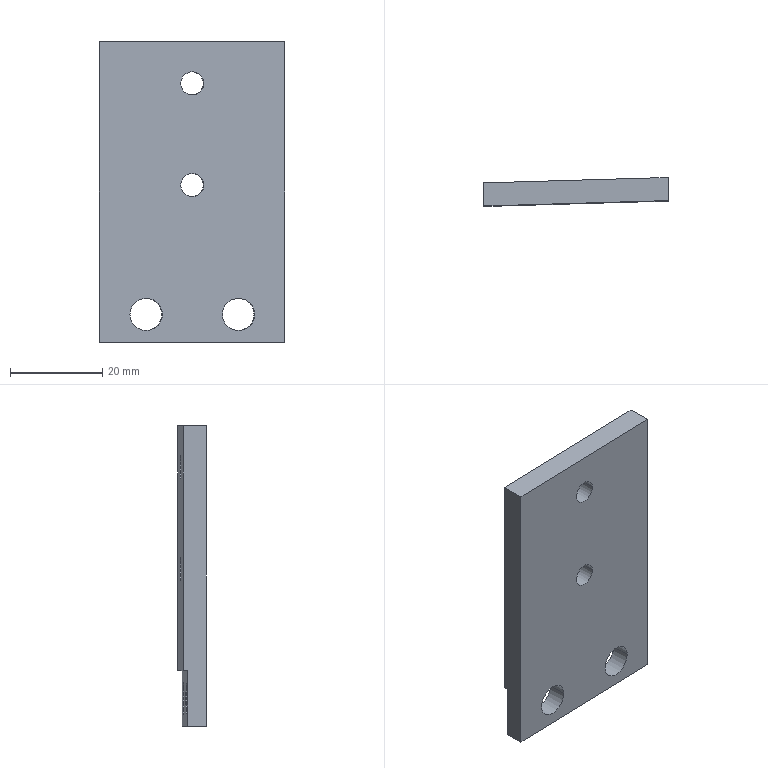Component | SolidWorks | CylinderFixingPlate2-1 | 1 solid | 16 faces | box 40.13 x 6.17 x 65 mm | volume 12016 mm3 | cylinder 8 | plane 8 | commonest cylinder face diameters 5 x4 7 x4 | material 6063
build123d program:
from build123d import *

# Parameters (mm, degrees)
SKETCH1_W             = 40
SKETCH1_H             = 65
BOSS_EXTRUDE1_DEPTH   = 2.5
SKETCH2_R             = 3.5
CUT_EXTRUDE1_DEPTH    = 39.487
M6_TAPPED_HOLE1_D     = 5
M6_TAPPED_HOLE1_DEPTH = 15
M6_TAPPED_HOLE1_TIP   = 1.502
SKETCH5_W             = 40
SKETCH5_H             = 12
CUT_EXTRUDE2_DEPTH    = 1


with BuildPart() as part:
    # Sketch1 → Boss-Extrude1 (new, symmetric)
    with BuildSketch(Plane.XY):
        Rectangle(SKETCH1_W, SKETCH1_H)
    extrude(amount=BOSS_EXTRUDE1_DEPTH, both=True)

    # Sketch2 → Cut-Extrude1 (cut, through all)
    with BuildSketch(Plane.XY.offset(2.5)):
        with Locations((10, 26.5)):
            Circle(SKETCH2_R)
        with Locations(Location((-10, 26.5, 0), (0, 0, 180))):
            Circle(SKETCH2_R)
    extrude(amount=-CUT_EXTRUDE1_DEPTH, mode=Mode.SUBTRACT)

    # M6 Tapped Hole1
    with Locations(Plane(origin=(0, -1.5, 2.5), x_dir=(1, 0, 0), z_dir=(0, 0, 1))):
        with Locations((0, 0), (0, -22)):
            Hole(M6_TAPPED_HOLE1_D / 2, depth=M6_TAPPED_HOLE1_DEPTH)
            with Locations((0, 0, -(M6_TAPPED_HOLE1_DEPTH + M6_TAPPED_HOLE1_TIP / 2))):  # 118° drill point
                Cone(0, M6_TAPPED_HOLE1_D / 2, M6_TAPPED_HOLE1_TIP, mode=Mode.SUBTRACT)

    # Sketch5 → Cut-Extrude2 (cut)
    with BuildSketch(Plane(origin=(0, 0, -2.5), x_dir=(-1, 0, 0), z_dir=(0, 0, -1))):
        with Locations((0, 26.5)):
            Rectangle(SKETCH5_W, SKETCH5_H)
    extrude(amount=-CUT_EXTRUDE2_DEPTH, mode=Mode.SUBTRACT)


solid = part.part

# Placed as in the assembly
solid = solid.moved(Location((191.273, -177.951, -1241.71), (90, 1.672, -180)))
STEP:
#1=COLOUR_RGB('',0.7922,0.8196,0.9333);
#2=FILL_AREA_STYLE_COLOUR('',#1);
#3=FILL_AREA_STYLE('',(#2));
#4=SURFACE_STYLE_FILL_AREA(#3);
#5=SURFACE_SIDE_STYLE('',(#4));
#6=SURFACE_STYLE_USAGE(.BOTH.,#5);
#7=PRESENTATION_STYLE_ASSIGNMENT((#6));
#8=CARTESIAN_POINT('',(7.626,-6.905,-48.827));
#9=VERTEX_POINT('',#8);
#10=CARTESIAN_POINT('',(7.429,-6.91,-48.827));
#11=VERTEX_POINT('',#10);
#12=CARTESIAN_POINT('',(7.528,-6.908,-48.827));
#13=DIRECTION('',(0.02918,-0.9996,-0.));
#14=DIRECTION('',(-0.9996,-0.02918,0.));
#15=AXIS2_PLACEMENT_3D('',#12,#13,#14);
#16=CIRCLE('',#15,0.09843);
#17=EDGE_CURVE('',#9,#11,#16,.T.);
#18=ORIENTED_EDGE('',*,*,#17,.F.);
#19=CARTESIAN_POINT('',(7.632,-7.101,-48.827));
#20=VERTEX_POINT('',#19);
#21=CARTESIAN_POINT('',(7.632,-7.101,-48.827));
#22=DIRECTION('',(0.02918,-0.9996,-0.));
#23=VECTOR('',#22,39.37);
#24=LINE('',#21,#23);
#25=EDGE_CURVE('',#9,#20,#24,.T.);
#26=ORIENTED_EDGE('',*,*,#25,.T.);
#27=CARTESIAN_POINT('',(7.435,-7.107,-48.827));
#28=VERTEX_POINT('',#27);
#29=CARTESIAN_POINT('',(7.533,-7.104,-48.827));
#30=DIRECTION('',(0.02918,-0.9996,-0.));
#31=DIRECTION('',(-0.9996,-0.02918,0.));
#32=AXIS2_PLACEMENT_3D('',#29,#30,#31);
#33=CIRCLE('',#32,0.09843);
#34=EDGE_CURVE('',#20,#28,#33,.T.);
#35=ORIENTED_EDGE('',*,*,#34,.T.);
#36=CARTESIAN_POINT('',(7.435,-7.107,-48.827));
#37=DIRECTION('',(0.02918,-0.9996,-0.));
#38=VECTOR('',#37,39.37);
#39=LINE('',#36,#38);
#40=EDGE_CURVE('',#11,#28,#39,.T.);
#41=ORIENTED_EDGE('',*,*,#40,.F.);
#42=EDGE_LOOP('',(#18,#26,#35,#41));
#43=FACE_OUTER_BOUND('',#42,.T.);
#44=CARTESIAN_POINT('',(7.533,-7.104,-48.827));
#45=DIRECTION('',(0.02918,-0.9996,-0.));
#46=DIRECTION('',(-0.9996,-0.02918,0.));
#47=AXIS2_PLACEMENT_3D('',#44,#45,#46);
#48=CYLINDRICAL_SURFACE('',#47,0.09843);
#49=ADVANCED_FACE('',(#43),#48,.F.);
#50=CARTESIAN_POINT('',(7.626,-6.905,-47.961));
#51=VERTEX_POINT('',#50);
#52=CARTESIAN_POINT('',(7.429,-6.91,-47.961));
#53=VERTEX_POINT('',#52);
#54=CARTESIAN_POINT('',(7.528,-6.908,-47.961));
#55=DIRECTION('',(0.02918,-0.9996,-0.));
#56=DIRECTION('',(-0.9996,-0.02918,0.));
#57=AXIS2_PLACEMENT_3D('',#54,#55,#56);
#58=CIRCLE('',#57,0.09843);
#59=EDGE_CURVE('',#51,#53,#58,.T.);
#60=ORIENTED_EDGE('',*,*,#59,.F.);
#61=CARTESIAN_POINT('',(7.632,-7.101,-47.961));
#62=VERTEX_POINT('',#61);
#63=CARTESIAN_POINT('',(7.632,-7.101,-47.961));
#64=DIRECTION('',(0.02918,-0.9996,-0.));
#65=VECTOR('',#64,39.37);
#66=LINE('',#63,#65);
#67=EDGE_CURVE('',#51,#62,#66,.T.);
#68=ORIENTED_EDGE('',*,*,#67,.T.);
#69=CARTESIAN_POINT('',(7.435,-7.107,-47.961));
#70=VERTEX_POINT('',#69);
#71=CARTESIAN_POINT('',(7.533,-7.104,-47.961));
#72=DIRECTION('',(0.02918,-0.9996,-0.));
#73=DIRECTION('',(-0.9996,-0.02918,0.));
#74=AXIS2_PLACEMENT_3D('',#71,#72,#73);
#75=CIRCLE('',#74,0.09843);
#76=EDGE_CURVE('',#62,#70,#75,.T.);
#77=ORIENTED_EDGE('',*,*,#76,.T.);
#78=CARTESIAN_POINT('',(7.435,-7.107,-47.961));
#79=DIRECTION('',(0.02918,-0.9996,-0.));
#80=VECTOR('',#79,39.37);
#81=LINE('',#78,#80);
#82=EDGE_CURVE('',#53,#70,#81,.T.);
#83=ORIENTED_EDGE('',*,*,#82,.F.);
#84=EDGE_LOOP('',(#60,#68,#77,#83));
#85=FACE_OUTER_BOUND('',#84,.T.);
#86=CARTESIAN_POINT('',(7.533,-7.104,-47.961));
#87=DIRECTION('',(0.02918,-0.9996,-0.));
#88=DIRECTION('',(-0.9996,-0.02918,0.));
#89=AXIS2_PLACEMENT_3D('',#86,#87,#88);
#90=CYLINDRICAL_SURFACE('',#89,0.09843);
#91=ADVANCED_FACE('',(#85),#90,.F.);
#92=CARTESIAN_POINT('',(8.06,-6.931,-49.93));
#93=VERTEX_POINT('',#92);
#94=CARTESIAN_POINT('',(7.785,-6.939,-49.93));
#95=VERTEX_POINT('',#94);
#96=CARTESIAN_POINT('',(7.922,-6.935,-49.93));
#97=DIRECTION('',(0.02918,-0.9996,-0.));
#98=DIRECTION('',(0.9996,0.02918,0.));
#99=AXIS2_PLACEMENT_3D('',#96,#97,#98);
#100=CIRCLE('',#99,0.1378);
#101=EDGE_CURVE('',#93,#95,#100,.T.);
#102=ORIENTED_EDGE('',*,*,#101,.F.);
#103=CARTESIAN_POINT('',(8.065,-7.089,-49.93));
#104=VERTEX_POINT('',#103);
#105=CARTESIAN_POINT('',(8.059,-6.892,-49.93));
#106=DIRECTION('',(0.02918,-0.9996,-0.));
#107=VECTOR('',#106,39.37);
#108=LINE('',#105,#107);
#109=EDGE_CURVE('',#93,#104,#108,.T.);
#110=ORIENTED_EDGE('',*,*,#109,.T.);
#111=CARTESIAN_POINT('',(7.789,-7.097,-49.93));
#112=VERTEX_POINT('',#111);
#113=CARTESIAN_POINT('',(7.927,-7.093,-49.93));
#114=DIRECTION('',(0.02918,-0.9996,-0.));
#115=DIRECTION('',(0.9996,0.02918,0.));
#116=AXIS2_PLACEMENT_3D('',#113,#114,#115);
#117=CIRCLE('',#116,0.1378);
#118=EDGE_CURVE('',#104,#112,#117,.T.);
#119=ORIENTED_EDGE('',*,*,#118,.T.);
#120=CARTESIAN_POINT('',(7.783,-6.9,-49.93));
#121=DIRECTION('',(0.02918,-0.9996,-0.));
#122=VECTOR('',#121,39.37);
#123=LINE('',#120,#122);
#124=EDGE_CURVE('',#95,#112,#123,.T.);
#125=ORIENTED_EDGE('',*,*,#124,.F.);
#126=EDGE_LOOP('',(#102,#110,#119,#125));
#127=FACE_OUTER_BOUND('',#126,.T.);
#128=CARTESIAN_POINT('',(7.921,-6.896,-49.93));
#129=DIRECTION('',(0.02918,-0.9996,-0.));
#130=DIRECTION('',(-0.9996,-0.02918,0.));
#131=AXIS2_PLACEMENT_3D('',#128,#129,#130);
#132=CYLINDRICAL_SURFACE('',#131,0.1378);
#133=ADVANCED_FACE('',(#127),#132,.F.);
#134=CARTESIAN_POINT('',(7.273,-6.954,-49.93));
#135=VERTEX_POINT('',#134);
#136=CARTESIAN_POINT('',(6.997,-6.962,-49.93));
#137=VERTEX_POINT('',#136);
#138=CARTESIAN_POINT('',(7.135,-6.958,-49.93));
#139=DIRECTION('',(0.02918,-0.9996,-0.));
#140=DIRECTION('',(0.9996,0.02918,0.));
#141=AXIS2_PLACEMENT_3D('',#138,#139,#140);
#142=CIRCLE('',#141,0.1378);
#143=EDGE_CURVE('',#135,#137,#142,.T.);
#144=ORIENTED_EDGE('',*,*,#143,.F.);
#145=CARTESIAN_POINT('',(7.278,-7.112,-49.93));
#146=VERTEX_POINT('',#145);
#147=CARTESIAN_POINT('',(7.272,-6.915,-49.93));
#148=DIRECTION('',(0.02918,-0.9996,-0.));
#149=VECTOR('',#148,39.37);
#150=LINE('',#147,#149);
#151=EDGE_CURVE('',#135,#146,#150,.T.);
#152=ORIENTED_EDGE('',*,*,#151,.T.);
#153=CARTESIAN_POINT('',(7.002,-7.12,-49.93));
#154=VERTEX_POINT('',#153);
#155=CARTESIAN_POINT('',(7.14,-7.116,-49.93));
#156=DIRECTION('',(0.02918,-0.9996,-0.));
#157=DIRECTION('',(-0.9996,-0.02918,0.));
#158=AXIS2_PLACEMENT_3D('',#155,#156,#157);
#159=CIRCLE('',#158,0.1378);
#160=EDGE_CURVE('',#146,#154,#159,.T.);
#161=ORIENTED_EDGE('',*,*,#160,.T.);
#162=CARTESIAN_POINT('',(6.996,-6.923,-49.93));
#163=DIRECTION('',(0.02918,-0.9996,-0.));
#164=VECTOR('',#163,39.37);
#165=LINE('',#162,#164);
#166=EDGE_CURVE('',#137,#154,#165,.T.);
#167=ORIENTED_EDGE('',*,*,#166,.F.);
#168=EDGE_LOOP('',(#144,#152,#161,#167));
#169=FACE_OUTER_BOUND('',#168,.T.);
#170=CARTESIAN_POINT('',(7.134,-6.919,-49.93));
#171=DIRECTION('',(0.02918,-0.9996,-0.));
#172=DIRECTION('',(-0.9996,-0.02918,0.));
#173=AXIS2_PLACEMENT_3D('',#170,#171,#172);
#174=CYLINDRICAL_SURFACE('',#173,0.1378);
#175=ADVANCED_FACE('',(#169),#174,.F.);
#176=CARTESIAN_POINT('',(8.316,-6.924,-50.166));
#177=VERTEX_POINT('',#176);
#178=CARTESIAN_POINT('',(6.742,-6.97,-50.166));
#179=VERTEX_POINT('',#178);
#180=CARTESIAN_POINT('',(6.742,-6.97,-50.166));
#181=DIRECTION('',(-0.9996,-0.02918,0.));
#182=VECTOR('',#181,39.37);
#183=LINE('',#180,#182);
#184=EDGE_CURVE('',#177,#179,#183,.T.);
#185=ORIENTED_EDGE('',*,*,#184,.F.);
#186=CARTESIAN_POINT('',(8.32,-7.081,-50.166));
#187=VERTEX_POINT('',#186);
#188=CARTESIAN_POINT('',(8.32,-7.081,-50.166));
#189=DIRECTION('',(-0.02918,0.9996,0.));
#190=VECTOR('',#189,39.37);
#191=LINE('',#188,#190);
#192=EDGE_CURVE('',#187,#177,#191,.T.);
#193=ORIENTED_EDGE('',*,*,#192,.F.);
#194=CARTESIAN_POINT('',(6.746,-7.127,-50.166));
#195=VERTEX_POINT('',#194);
#196=CARTESIAN_POINT('',(8.32,-7.081,-50.166));
#197=DIRECTION('',(0.9996,0.02918,-0.));
#198=VECTOR('',#197,39.37);
#199=LINE('',#196,#198);
#200=EDGE_CURVE('',#195,#187,#199,.T.);
#201=ORIENTED_EDGE('',*,*,#200,.F.);
#202=CARTESIAN_POINT('',(6.746,-7.127,-50.166));
#203=DIRECTION('',(-0.02918,0.9996,0.));
#204=VECTOR('',#203,39.37);
#205=LINE('',#202,#204);
#206=EDGE_CURVE('',#195,#179,#205,.T.);
#207=ORIENTED_EDGE('',*,*,#206,.T.);
#208=EDGE_LOOP('',(#185,#193,#201,#207));
#209=FACE_OUTER_BOUND('',#208,.T.);
#210=CARTESIAN_POINT('',(8.32,-7.081,-50.166));
#211=DIRECTION('',(0.,-0.,1.));
#212=DIRECTION('',(-0.02918,0.9996,0.));
#213=AXIS2_PLACEMENT_3D('',#210,#211,#212);
#214=PLANE('',#213);
#215=ADVANCED_FACE('',(#209),#214,.F.);
#216=ORIENTED_EDGE('',*,*,#151,.F.);
#217=CARTESIAN_POINT('',(7.135,-6.958,-49.93));
#218=DIRECTION('',(0.02918,-0.9996,-0.));
#219=DIRECTION('',(0.9996,0.02918,0.));
#220=AXIS2_PLACEMENT_3D('',#217,#218,#219);
#221=CIRCLE('',#220,0.1378);
#222=EDGE_CURVE('',#137,#135,#221,.T.);
#223=ORIENTED_EDGE('',*,*,#222,.F.);
#224=ORIENTED_EDGE('',*,*,#166,.T.);
#225=CARTESIAN_POINT('',(7.14,-7.116,-49.93));
#226=DIRECTION('',(0.02918,-0.9996,-0.));
#227=DIRECTION('',(-0.9996,-0.02918,0.));
#228=AXIS2_PLACEMENT_3D('',#225,#226,#227);
#229=CIRCLE('',#228,0.1378);
#230=EDGE_CURVE('',#154,#146,#229,.T.);
#231=ORIENTED_EDGE('',*,*,#230,.T.);
#232=EDGE_LOOP('',(#216,#223,#224,#231));
#233=FACE_OUTER_BOUND('',#232,.T.);
#234=CARTESIAN_POINT('',(7.134,-6.919,-49.93));
#235=DIRECTION('',(0.02918,-0.9996,-0.));
#236=DIRECTION('',(-0.9996,-0.02918,0.));
#237=AXIS2_PLACEMENT_3D('',#234,#235,#236);
#238=CYLINDRICAL_SURFACE('',#237,0.1378);
#239=ADVANCED_FACE('',(#233),#238,.F.);
#240=ORIENTED_EDGE('',*,*,#109,.F.);
#241=CARTESIAN_POINT('',(7.922,-6.935,-49.93));
#242=DIRECTION('',(0.02918,-0.9996,-0.));
#243=DIRECTION('',(0.9996,0.02918,0.));
#244=AXIS2_PLACEMENT_3D('',#241,#242,#243);
#245=CIRCLE('',#244,0.1378);
#246=EDGE_CURVE('',#95,#93,#245,.T.);
#247=ORIENTED_EDGE('',*,*,#246,.F.);
#248=ORIENTED_EDGE('',*,*,#124,.T.);
#249=CARTESIAN_POINT('',(7.927,-7.093,-49.93));
#250=DIRECTION('',(0.02918,-0.9996,-0.));
#251=DIRECTION('',(0.9996,0.02918,0.));
#252=AXIS2_PLACEMENT_3D('',#249,#250,#251);
#253=CIRCLE('',#252,0.1378);
#254=EDGE_CURVE('',#112,#104,#253,.T.);
#255=ORIENTED_EDGE('',*,*,#254,.T.);
#256=EDGE_LOOP('',(#240,#247,#248,#255));
#257=FACE_OUTER_BOUND('',#256,.T.);
#258=CARTESIAN_POINT('',(7.921,-6.896,-49.93));
#259=DIRECTION('',(0.02918,-0.9996,-0.));
#260=DIRECTION('',(-0.9996,-0.02918,0.));
#261=AXIS2_PLACEMENT_3D('',#258,#259,#260);
#262=CYLINDRICAL_SURFACE('',#261,0.1378);
#263=ADVANCED_FACE('',(#257),#262,.F.);
#264=CARTESIAN_POINT('',(6.74,-6.931,-47.607));
#265=VERTEX_POINT('',#264);
#266=CARTESIAN_POINT('',(6.74,-6.931,-49.693));
#267=VERTEX_POINT('',#266);
#268=CARTESIAN_POINT('',(6.74,-6.931,-50.166));
#269=DIRECTION('',(-0.,0.,-1.));
#270=VECTOR('',#269,39.37);
#271=LINE('',#268,#270);
#272=EDGE_CURVE('',#265,#267,#271,.T.);
#273=ORIENTED_EDGE('',*,*,#272,.T.);
#274=CARTESIAN_POINT('',(6.742,-6.97,-49.693));
#275=VERTEX_POINT('',#274);
#276=CARTESIAN_POINT('',(6.742,-6.97,-49.693));
#277=DIRECTION('',(-0.02918,0.9996,0.));
#278=VECTOR('',#277,39.37);
#279=LINE('',#276,#278);
#280=EDGE_CURVE('',#275,#267,#279,.T.);
#281=ORIENTED_EDGE('',*,*,#280,.F.);
#282=CARTESIAN_POINT('',(6.742,-6.97,-50.166));
#283=DIRECTION('',(0.,-0.,1.));
#284=VECTOR('',#283,39.37);
#285=LINE('',#282,#284);
#286=EDGE_CURVE('',#179,#275,#285,.T.);
#287=ORIENTED_EDGE('',*,*,#286,.F.);
#288=ORIENTED_EDGE('',*,*,#206,.F.);
#289=CARTESIAN_POINT('',(6.746,-7.127,-47.607));
#290=VERTEX_POINT('',#289);
#291=CARTESIAN_POINT('',(6.746,-7.127,-50.166));
#292=DIRECTION('',(-0.,0.,-1.));
#293=VECTOR('',#292,39.37);
#294=LINE('',#291,#293);
#295=EDGE_CURVE('',#290,#195,#294,.T.);
#296=ORIENTED_EDGE('',*,*,#295,.F.);
#297=CARTESIAN_POINT('',(6.746,-7.127,-47.607));
#298=DIRECTION('',(-0.02918,0.9996,0.));
#299=VECTOR('',#298,39.37);
#300=LINE('',#297,#299);
#301=EDGE_CURVE('',#290,#265,#300,.T.);
#302=ORIENTED_EDGE('',*,*,#301,.T.);
#303=EDGE_LOOP('',(#273,#281,#287,#288,#296,#302));
#304=FACE_OUTER_BOUND('',#303,.T.);
#305=CARTESIAN_POINT('',(6.746,-7.127,-50.166));
#306=DIRECTION('',(0.9996,0.02918,-0.));
#307=DIRECTION('',(0.,-0.,1.));
#308=AXIS2_PLACEMENT_3D('',#305,#306,#307);
#309=PLANE('',#308);
#310=ADVANCED_FACE('',(#304),#309,.F.);
#311=CARTESIAN_POINT('',(8.316,-6.924,-49.693));
#312=VERTEX_POINT('',#311);
#313=CARTESIAN_POINT('',(8.316,-6.924,-50.166));
#314=DIRECTION('',(-0.,0.,-1.));
#315=VECTOR('',#314,39.37);
#316=LINE('',#313,#315);
#317=EDGE_CURVE('',#312,#177,#316,.T.);
#318=ORIENTED_EDGE('',*,*,#317,.F.);
#319=CARTESIAN_POINT('',(8.315,-6.885,-49.693));
#320=VERTEX_POINT('',#319);
#321=CARTESIAN_POINT('',(8.316,-6.924,-49.693));
#322=DIRECTION('',(-0.02918,0.9996,0.));
#323=VECTOR('',#322,39.37);
#324=LINE('',#321,#323);
#325=EDGE_CURVE('',#312,#320,#324,.T.);
#326=ORIENTED_EDGE('',*,*,#325,.T.);
#327=CARTESIAN_POINT('',(8.315,-6.885,-47.607));
#328=VERTEX_POINT('',#327);
#329=CARTESIAN_POINT('',(8.315,-6.885,-50.166));
#330=DIRECTION('',(0.,-0.,1.));
#331=VECTOR('',#330,39.37);
#332=LINE('',#329,#331);
#333=EDGE_CURVE('',#320,#328,#332,.T.);
#334=ORIENTED_EDGE('',*,*,#333,.T.);
#335=CARTESIAN_POINT('',(8.32,-7.081,-47.607));
#336=VERTEX_POINT('',#335);
#337=CARTESIAN_POINT('',(8.32,-7.081,-47.607));
#338=DIRECTION('',(-0.02918,0.9996,0.));
#339=VECTOR('',#338,39.37);
#340=LINE('',#337,#339);
#341=EDGE_CURVE('',#336,#328,#340,.T.);
#342=ORIENTED_EDGE('',*,*,#341,.F.);
#343=CARTESIAN_POINT('',(8.32,-7.081,-50.166));
#344=DIRECTION('',(0.,-0.,1.));
#345=VECTOR('',#344,39.37);
#346=LINE('',#343,#345);
#347=EDGE_CURVE('',#187,#336,#346,.T.);
#348=ORIENTED_EDGE('',*,*,#347,.F.);
#349=ORIENTED_EDGE('',*,*,#192,.T.);
#350=EDGE_LOOP('',(#318,#326,#334,#342,#348,#349));
#351=FACE_OUTER_BOUND('',#350,.T.);
#352=CARTESIAN_POINT('',(8.32,-7.081,-50.166));
#353=DIRECTION('',(-0.9996,-0.02918,0.));
#354=DIRECTION('',(-0.,0.,-1.));
#355=AXIS2_PLACEMENT_3D('',#352,#353,#354);
#356=PLANE('',#355);
#357=ADVANCED_FACE('',(#351),#356,.F.);
#358=CARTESIAN_POINT('',(8.315,-6.885,-47.607));
#359=DIRECTION('',(-0.9996,-0.02918,0.));
#360=VECTOR('',#359,39.37);
#361=LINE('',#358,#360);
#362=EDGE_CURVE('',#328,#265,#361,.T.);
#363=ORIENTED_EDGE('',*,*,#362,.T.);
#364=ORIENTED_EDGE('',*,*,#301,.F.);
#365=CARTESIAN_POINT('',(8.32,-7.081,-47.607));
#366=DIRECTION('',(-0.9996,-0.02918,0.));
#367=VECTOR('',#366,39.37);
#368=LINE('',#365,#367);
#369=EDGE_CURVE('',#336,#290,#368,.T.);
#370=ORIENTED_EDGE('',*,*,#369,.F.);
#371=ORIENTED_EDGE('',*,*,#341,.T.);
#372=EDGE_LOOP('',(#363,#364,#370,#371));
#373=FACE_OUTER_BOUND('',#372,.T.);
#374=CARTESIAN_POINT('',(8.32,-7.081,-47.607));
#375=DIRECTION('',(-0.,0.,-1.));
#376=DIRECTION('',(0.02918,-0.9996,-0.));
#377=AXIS2_PLACEMENT_3D('',#374,#375,#376);
#378=PLANE('',#377);
#379=ADVANCED_FACE('',(#373),#378,.F.);
#380=CARTESIAN_POINT('',(7.533,-7.104,-48.827));
#381=DIRECTION('',(0.02918,-0.9996,-0.));
#382=DIRECTION('',(-0.9996,-0.02918,0.));
#383=AXIS2_PLACEMENT_3D('',#380,#381,#382);
#384=CIRCLE('',#383,0.09843);
#385=EDGE_CURVE('',#28,#20,#384,.T.);
#386=ORIENTED_EDGE('',*,*,#385,.F.);
#387=ORIENTED_EDGE('',*,*,#34,.F.);
#388=EDGE_LOOP('',(#386,#387));
#389=FACE_BOUND('',#388,.T.);
#390=CARTESIAN_POINT('',(7.533,-7.104,-47.961));
#391=DIRECTION('',(0.02918,-0.9996,-0.));
#392=DIRECTION('',(-0.9996,-0.02918,0.));
#393=AXIS2_PLACEMENT_3D('',#390,#391,#392);
#394=CIRCLE('',#393,0.09843);
#395=EDGE_CURVE('',#70,#62,#394,.T.);
#396=ORIENTED_EDGE('',*,*,#395,.F.);
#397=ORIENTED_EDGE('',*,*,#76,.F.);
#398=EDGE_LOOP('',(#396,#397));
#399=FACE_BOUND('',#398,.T.);
#400=ORIENTED_EDGE('',*,*,#254,.F.);
#401=ORIENTED_EDGE('',*,*,#118,.F.);
#402=EDGE_LOOP('',(#400,#401));
#403=FACE_BOUND('',#402,.T.);
#404=ORIENTED_EDGE('',*,*,#230,.F.);
#405=ORIENTED_EDGE('',*,*,#160,.F.);
#406=EDGE_LOOP('',(#404,#405));
#407=FACE_BOUND('',#406,.T.);
#408=ORIENTED_EDGE('',*,*,#295,.T.);
#409=ORIENTED_EDGE('',*,*,#200,.T.);
#410=ORIENTED_EDGE('',*,*,#347,.T.);
#411=ORIENTED_EDGE('',*,*,#369,.T.);
#412=EDGE_LOOP('',(#408,#409,#410,#411));
#413=FACE_OUTER_BOUND('',#412,.T.);
#414=CARTESIAN_POINT('',(7.533,-7.104,-48.886));
#415=DIRECTION('',(0.02918,-0.9996,-0.));
#416=DIRECTION('',(-0.9996,-0.02918,0.));
#417=AXIS2_PLACEMENT_3D('',#414,#415,#416);
#418=PLANE('',#417);
#419=ADVANCED_FACE('',(#389,#399,#403,#407,#413),#418,.T.);
#420=CARTESIAN_POINT('',(7.528,-6.908,-48.827));
#421=DIRECTION('',(0.02918,-0.9996,-0.));
#422=DIRECTION('',(-0.9996,-0.02918,0.));
#423=AXIS2_PLACEMENT_3D('',#420,#421,#422);
#424=CIRCLE('',#423,0.09843);
#425=EDGE_CURVE('',#11,#9,#424,.T.);
#426=ORIENTED_EDGE('',*,*,#425,.T.);
#427=ORIENTED_EDGE('',*,*,#17,.T.);
#428=EDGE_LOOP('',(#426,#427));
#429=FACE_BOUND('',#428,.T.);
#430=CARTESIAN_POINT('',(7.528,-6.908,-47.961));
#431=DIRECTION('',(0.02918,-0.9996,-0.));
#432=DIRECTION('',(-0.9996,-0.02918,0.));
#433=AXIS2_PLACEMENT_3D('',#430,#431,#432);
#434=CIRCLE('',#433,0.09843);
#435=EDGE_CURVE('',#53,#51,#434,.T.);
#436=ORIENTED_EDGE('',*,*,#435,.T.);
#437=ORIENTED_EDGE('',*,*,#59,.T.);
#438=EDGE_LOOP('',(#436,#437));
#439=FACE_BOUND('',#438,.T.);
#440=ORIENTED_EDGE('',*,*,#333,.F.);
#441=CARTESIAN_POINT('',(6.74,-6.931,-49.693));
#442=DIRECTION('',(0.9996,0.02918,-0.));
#443=VECTOR('',#442,39.37);
#444=LINE('',#441,#443);
#445=EDGE_CURVE('',#267,#320,#444,.T.);
#446=ORIENTED_EDGE('',*,*,#445,.F.);
#447=ORIENTED_EDGE('',*,*,#272,.F.);
#448=ORIENTED_EDGE('',*,*,#362,.F.);
#449=EDGE_LOOP('',(#440,#446,#447,#448));
#450=FACE_OUTER_BOUND('',#449,.T.);
#451=CARTESIAN_POINT('',(7.528,-6.908,-48.886));
#452=DIRECTION('',(0.02918,-0.9996,-0.));
#453=DIRECTION('',(-0.9996,-0.02918,0.));
#454=AXIS2_PLACEMENT_3D('',#451,#452,#453);
#455=PLANE('',#454);
#456=ADVANCED_FACE('',(#429,#439,#450),#455,.F.);
#457=ORIENTED_EDGE('',*,*,#67,.F.);
#458=ORIENTED_EDGE('',*,*,#435,.F.);
#459=ORIENTED_EDGE('',*,*,#82,.T.);
#460=ORIENTED_EDGE('',*,*,#395,.T.);
#461=EDGE_LOOP('',(#457,#458,#459,#460));
#462=FACE_OUTER_BOUND('',#461,.T.);
#463=CARTESIAN_POINT('',(7.533,-7.104,-47.961));
#464=DIRECTION('',(0.02918,-0.9996,-0.));
#465=DIRECTION('',(-0.9996,-0.02918,0.));
#466=AXIS2_PLACEMENT_3D('',#463,#464,#465);
#467=CYLINDRICAL_SURFACE('',#466,0.09843);
#468=ADVANCED_FACE('',(#462),#467,.F.);
#469=ORIENTED_EDGE('',*,*,#25,.F.);
#470=ORIENTED_EDGE('',*,*,#425,.F.);
#471=ORIENTED_EDGE('',*,*,#40,.T.);
#472=ORIENTED_EDGE('',*,*,#385,.T.);
#473=EDGE_LOOP('',(#469,#470,#471,#472));
#474=FACE_OUTER_BOUND('',#473,.T.);
#475=CARTESIAN_POINT('',(7.533,-7.104,-48.827));
#476=DIRECTION('',(0.02918,-0.9996,-0.));
#477=DIRECTION('',(-0.9996,-0.02918,0.));
#478=AXIS2_PLACEMENT_3D('',#475,#476,#477);
#479=CYLINDRICAL_SURFACE('',#478,0.09843);
#480=ADVANCED_FACE('',(#474),#479,.F.);
#481=ORIENTED_EDGE('',*,*,#246,.T.);
#482=ORIENTED_EDGE('',*,*,#101,.T.);
#483=EDGE_LOOP('',(#481,#482));
#484=FACE_BOUND('',#483,.T.);
#485=ORIENTED_EDGE('',*,*,#286,.T.);
#486=CARTESIAN_POINT('',(6.742,-6.97,-49.693));
#487=DIRECTION('',(0.9996,0.02918,-0.));
#488=VECTOR('',#487,39.37);
#489=LINE('',#486,#488);
#490=EDGE_CURVE('',#275,#312,#489,.T.);
#491=ORIENTED_EDGE('',*,*,#490,.T.);
#492=ORIENTED_EDGE('',*,*,#317,.T.);
#493=ORIENTED_EDGE('',*,*,#184,.T.);
#494=EDGE_LOOP('',(#485,#491,#492,#493));
#495=FACE_OUTER_BOUND('',#494,.T.);
#496=ORIENTED_EDGE('',*,*,#222,.T.);
#497=ORIENTED_EDGE('',*,*,#143,.T.);
#498=EDGE_LOOP('',(#496,#497));
#499=FACE_BOUND('',#498,.T.);
#500=CARTESIAN_POINT('',(7.529,-6.947,-48.886));
#501=DIRECTION('',(-0.02918,0.9996,0.));
#502=DIRECTION('',(0.9996,0.02918,-0.));
#503=AXIS2_PLACEMENT_3D('',#500,#501,#502);
#504=PLANE('',#503);
#505=ADVANCED_FACE('',(#484,#495,#499),#504,.T.);
#506=ORIENTED_EDGE('',*,*,#445,.T.);
#507=ORIENTED_EDGE('',*,*,#325,.F.);
#508=ORIENTED_EDGE('',*,*,#490,.F.);
#509=ORIENTED_EDGE('',*,*,#280,.T.);
#510=EDGE_LOOP('',(#506,#507,#508,#509));
#511=FACE_OUTER_BOUND('',#510,.T.);
#512=CARTESIAN_POINT('',(6.742,-6.97,-49.693));
#513=DIRECTION('',(0.,-0.,1.));
#514=DIRECTION('',(-0.02918,0.9996,0.));
#515=AXIS2_PLACEMENT_3D('',#512,#513,#514);
#516=PLANE('',#515);
#517=ADVANCED_FACE('',(#511),#516,.F.);
#518=CLOSED_SHELL('',(#49,#91,#133,#175,#215,#239,#263,#310,#357,#379,#419,#456,#468,#480,#505,#517));
#519=MANIFOLD_SOLID_BREP('',#518);
#520=STYLED_ITEM('',(#7),#519);
#521=(LENGTH_UNIT()NAMED_UNIT(*)SI_UNIT($,.METRE.));
#522=LENGTH_MEASURE_WITH_UNIT(LENGTH_MEASURE(0.0254),#521);
#523=DIMENSIONAL_EXPONENTS(1.,0.,0.,0.,0.,0.,0.);
#524=(CONVERSION_BASED_UNIT('',#522)LENGTH_UNIT()NAMED_UNIT(#523));
#525=UNCERTAINTY_MEASURE_WITH_UNIT(LENGTH_MEASURE(0.00001),#524,'','');
#526=(NAMED_UNIT(*)PLANE_ANGLE_UNIT()SI_UNIT($,.RADIAN.));
#527=(NAMED_UNIT(*)SI_UNIT($,.STERADIAN.)SOLID_ANGLE_UNIT());
#528=(GEOMETRIC_REPRESENTATION_CONTEXT(3)GLOBAL_UNCERTAINTY_ASSIGNED_CONTEXT((#525))GLOBAL_UNIT_ASSIGNED_CONTEXT((#524,#526,#527))REPRESENTATION_CONTEXT('',''));
#529=MECHANICAL_DESIGN_GEOMETRIC_PRESENTATION_REPRESENTATION('',(#520),#528);
#530=CARTESIAN_POINT('',(0.,0.,0.));
#531=DIRECTION('',(0.,0.,1.));
#532=DIRECTION('',(1.,0.,0.));
#533=AXIS2_PLACEMENT_3D('',#530,#531,#532);
#534=(LENGTH_UNIT()NAMED_UNIT(*)SI_UNIT($,.METRE.));
#535=LENGTH_MEASURE_WITH_UNIT(LENGTH_MEASURE(0.0254),#534);
#536=DIMENSIONAL_EXPONENTS(1.,0.,0.,0.,0.,0.,0.);
#537=(CONVERSION_BASED_UNIT('',#535)LENGTH_UNIT()NAMED_UNIT(#536));
#538=UNCERTAINTY_MEASURE_WITH_UNIT(LENGTH_MEASURE(0.00001),#537,'','');
#539=(NAMED_UNIT(*)PLANE_ANGLE_UNIT()SI_UNIT($,.RADIAN.));
#540=(NAMED_UNIT(*)SI_UNIT($,.STERADIAN.)SOLID_ANGLE_UNIT());
#541=(GEOMETRIC_REPRESENTATION_CONTEXT(3)GLOBAL_UNCERTAINTY_ASSIGNED_CONTEXT((#538))GLOBAL_UNIT_ASSIGNED_CONTEXT((#537,#539,#540))REPRESENTATION_CONTEXT('',''));
#542=ADVANCED_BREP_SHAPE_REPRESENTATION('',(#519,#533),#541);
#543=PRESENTATION_LAYER_ASSIGNMENT('','',(#520));